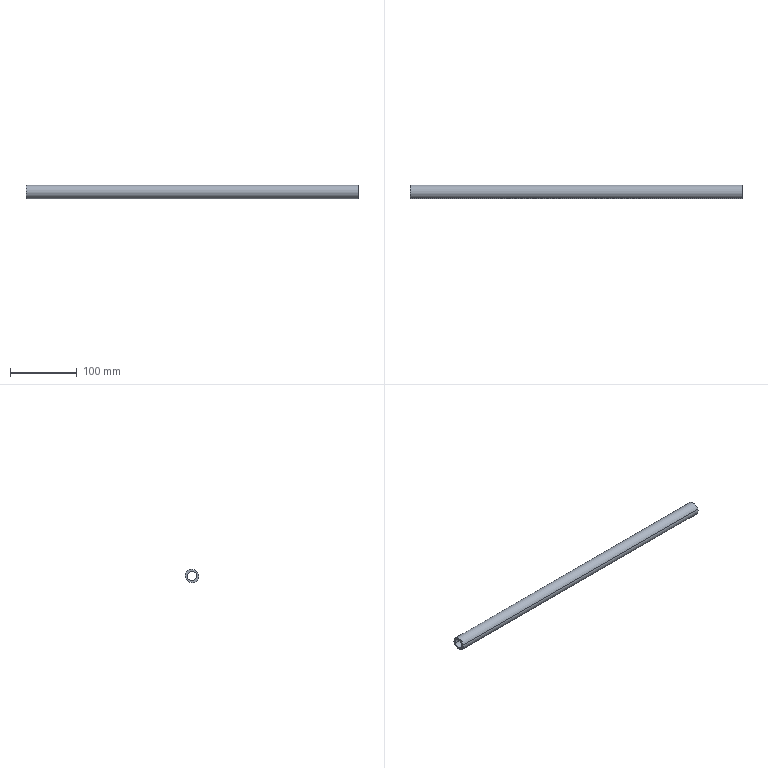Component | SolidWorks | Part9-1 | 1 solid | 6 faces | box 498 x 20 x 20 mm | volume 79790 mm3 | cylinder 4 | plane 2 | commonest cylinder face diameters 14 x2 20 x2 | material 45
build123d program:
from build123d import *

# Parameters (mm, degrees)
BOSS_EXTRUDE1_DEPTH      = 462
BOSS_EXTRUDE1_DEPTH_BACK = 36
SKETCH4_R                = 10
SKETCH5_R                = 7
CUT_EXTRUDE1_DEPTH       = 500.106


with BuildPart() as part:
    # Sketch4 → Boss-Extrude1 (new, two sides: drawn at the far end of the back side and taken through both)
    with BuildSketch(Plane.XY.offset(-BOSS_EXTRUDE1_DEPTH_BACK)):
        with Locations((16.5, -10.004)):
            Circle(SKETCH4_R)
    extrude(amount=BOSS_EXTRUDE1_DEPTH + BOSS_EXTRUDE1_DEPTH_BACK)

    # Sketch5 → Cut-Extrude1 (cut, through all)
    with BuildSketch(Plane(origin=(0, 0, -36), x_dir=(-1, 0, 0), z_dir=(0, 0, -1))):
        with Locations((-16.5, -10.004)):
            Circle(SKETCH5_R)
    extrude(amount=-CUT_EXTRUDE1_DEPTH, mode=Mode.SUBTRACT)


solid = part.part

# Placed as in the assembly
solid = solid.moved(Location((8.954, -34.996, 26.504), (0, 90, 0)))
STEP:
#1=CARTESIAN_POINT('',(18.541,-2.036,0.4706));
#2=VERTEX_POINT('',#1);
#3=CARTESIAN_POINT('',(18.541,-1.507,0.3171));
#4=VERTEX_POINT('',#3);
#5=CARTESIAN_POINT('',(18.541,-1.772,0.3939));
#6=DIRECTION('',(-1.,-0.,0.));
#7=DIRECTION('',(0.,0.9604,-0.2785));
#8=AXIS2_PLACEMENT_3D('',#5,#6,#7);
#9=CIRCLE('',#8,0.2756);
#10=EDGE_CURVE('',#2,#4,#9,.T.);
#11=ORIENTED_EDGE('',*,*,#10,.F.);
#12=CARTESIAN_POINT('',(-1.065,-2.036,0.4706));
#13=VERTEX_POINT('',#12);
#14=CARTESIAN_POINT('',(18.541,-2.036,0.4706));
#15=DIRECTION('',(-1.,-0.,0.));
#16=VECTOR('',#15,39.37);
#17=LINE('',#14,#16);
#18=EDGE_CURVE('',#2,#13,#17,.T.);
#19=ORIENTED_EDGE('',*,*,#18,.T.);
#20=CARTESIAN_POINT('',(-1.065,-1.507,0.3171));
#21=VERTEX_POINT('',#20);
#22=CARTESIAN_POINT('',(-1.065,-1.772,0.3939));
#23=DIRECTION('',(-1.,-0.,0.));
#24=DIRECTION('',(0.,0.9604,-0.2785));
#25=AXIS2_PLACEMENT_3D('',#22,#23,#24);
#26=CIRCLE('',#25,0.2756);
#27=EDGE_CURVE('',#13,#21,#26,.T.);
#28=ORIENTED_EDGE('',*,*,#27,.T.);
#29=CARTESIAN_POINT('',(18.541,-1.507,0.3171));
#30=DIRECTION('',(-1.,-0.,0.));
#31=VECTOR('',#30,39.37);
#32=LINE('',#29,#31);
#33=EDGE_CURVE('',#4,#21,#32,.T.);
#34=ORIENTED_EDGE('',*,*,#33,.F.);
#35=EDGE_LOOP('',(#11,#19,#28,#34));
#36=FACE_OUTER_BOUND('',#35,.T.);
#37=CARTESIAN_POINT('',(18.541,-1.772,0.3939));
#38=DIRECTION('',(-1.,-0.,0.));
#39=DIRECTION('',(0.,0.9604,-0.2785));
#40=AXIS2_PLACEMENT_3D('',#37,#38,#39);
#41=CYLINDRICAL_SURFACE('',#40,0.2756);
#42=ADVANCED_FACE('',(#36),#41,.F.);
#43=CARTESIAN_POINT('',(-1.065,-2.15,0.5035));
#44=VERTEX_POINT('',#43);
#45=CARTESIAN_POINT('',(-1.065,-1.394,0.2842));
#46=VERTEX_POINT('',#45);
#47=CARTESIAN_POINT('',(-1.065,-1.772,0.3939));
#48=DIRECTION('',(1.,0.,-0.));
#49=DIRECTION('',(0.,-0.9604,0.2785));
#50=AXIS2_PLACEMENT_3D('',#47,#48,#49);
#51=CIRCLE('',#50,0.3937);
#52=EDGE_CURVE('',#44,#46,#51,.T.);
#53=ORIENTED_EDGE('',*,*,#52,.T.);
#54=CARTESIAN_POINT('',(18.541,-1.394,0.2842));
#55=VERTEX_POINT('',#54);
#56=CARTESIAN_POINT('',(-1.065,-1.394,0.2842));
#57=DIRECTION('',(1.,0.,-0.));
#58=VECTOR('',#57,39.37);
#59=LINE('',#56,#58);
#60=EDGE_CURVE('',#46,#55,#59,.T.);
#61=ORIENTED_EDGE('',*,*,#60,.T.);
#62=CARTESIAN_POINT('',(18.541,-2.15,0.5035));
#63=VERTEX_POINT('',#62);
#64=CARTESIAN_POINT('',(18.541,-1.772,0.3939));
#65=DIRECTION('',(1.,0.,-0.));
#66=DIRECTION('',(0.,-0.9604,0.2785));
#67=AXIS2_PLACEMENT_3D('',#64,#65,#66);
#68=CIRCLE('',#67,0.3937);
#69=EDGE_CURVE('',#63,#55,#68,.T.);
#70=ORIENTED_EDGE('',*,*,#69,.F.);
#71=CARTESIAN_POINT('',(-1.065,-2.15,0.5035));
#72=DIRECTION('',(1.,0.,-0.));
#73=VECTOR('',#72,39.37);
#74=LINE('',#71,#73);
#75=EDGE_CURVE('',#44,#63,#74,.T.);
#76=ORIENTED_EDGE('',*,*,#75,.F.);
#77=EDGE_LOOP('',(#53,#61,#70,#76));
#78=FACE_OUTER_BOUND('',#77,.T.);
#79=CARTESIAN_POINT('',(-1.065,-1.772,0.3939));
#80=DIRECTION('',(1.,0.,-0.));
#81=DIRECTION('',(0.,-0.9604,0.2785));
#82=AXIS2_PLACEMENT_3D('',#79,#80,#81);
#83=CYLINDRICAL_SURFACE('',#82,0.3937);
#84=ADVANCED_FACE('',(#78),#83,.T.);
#85=ORIENTED_EDGE('',*,*,#60,.F.);
#86=CARTESIAN_POINT('',(-1.065,-1.772,0.3939));
#87=DIRECTION('',(1.,0.,-0.));
#88=DIRECTION('',(0.,-0.9604,0.2785));
#89=AXIS2_PLACEMENT_3D('',#86,#87,#88);
#90=CIRCLE('',#89,0.3937);
#91=EDGE_CURVE('',#46,#44,#90,.T.);
#92=ORIENTED_EDGE('',*,*,#91,.T.);
#93=ORIENTED_EDGE('',*,*,#75,.T.);
#94=CARTESIAN_POINT('',(18.541,-1.772,0.3939));
#95=DIRECTION('',(1.,0.,-0.));
#96=DIRECTION('',(0.,-0.9604,0.2785));
#97=AXIS2_PLACEMENT_3D('',#94,#95,#96);
#98=CIRCLE('',#97,0.3937);
#99=EDGE_CURVE('',#55,#63,#98,.T.);
#100=ORIENTED_EDGE('',*,*,#99,.F.);
#101=EDGE_LOOP('',(#85,#92,#93,#100));
#102=FACE_OUTER_BOUND('',#101,.T.);
#103=CARTESIAN_POINT('',(-1.065,-1.772,0.3939));
#104=DIRECTION('',(1.,0.,-0.));
#105=DIRECTION('',(0.,-0.9604,0.2785));
#106=AXIS2_PLACEMENT_3D('',#103,#104,#105);
#107=CYLINDRICAL_SURFACE('',#106,0.3937);
#108=ADVANCED_FACE('',(#102),#107,.T.);
#109=CARTESIAN_POINT('',(-1.065,-1.772,0.3939));
#110=DIRECTION('',(-1.,-0.,0.));
#111=DIRECTION('',(0.,0.9604,-0.2785));
#112=AXIS2_PLACEMENT_3D('',#109,#110,#111);
#113=CIRCLE('',#112,0.2756);
#114=EDGE_CURVE('',#21,#13,#113,.T.);
#115=ORIENTED_EDGE('',*,*,#114,.F.);
#116=ORIENTED_EDGE('',*,*,#27,.F.);
#117=EDGE_LOOP('',(#115,#116));
#118=FACE_BOUND('',#117,.T.);
#119=ORIENTED_EDGE('',*,*,#52,.F.);
#120=ORIENTED_EDGE('',*,*,#91,.F.);
#121=EDGE_LOOP('',(#119,#120));
#122=FACE_OUTER_BOUND('',#121,.T.);
#123=CARTESIAN_POINT('',(-1.065,-1.772,0.3939));
#124=DIRECTION('',(1.,0.,-0.));
#125=DIRECTION('',(0.,-0.9604,0.2785));
#126=AXIS2_PLACEMENT_3D('',#123,#124,#125);
#127=PLANE('',#126);
#128=ADVANCED_FACE('',(#118,#122),#127,.F.);
#129=CARTESIAN_POINT('',(18.541,-1.772,0.3939));
#130=DIRECTION('',(-1.,-0.,0.));
#131=DIRECTION('',(0.,0.9604,-0.2785));
#132=AXIS2_PLACEMENT_3D('',#129,#130,#131);
#133=CIRCLE('',#132,0.2756);
#134=EDGE_CURVE('',#4,#2,#133,.T.);
#135=ORIENTED_EDGE('',*,*,#134,.T.);
#136=ORIENTED_EDGE('',*,*,#10,.T.);
#137=EDGE_LOOP('',(#135,#136));
#138=FACE_BOUND('',#137,.T.);
#139=ORIENTED_EDGE('',*,*,#69,.T.);
#140=ORIENTED_EDGE('',*,*,#99,.T.);
#141=EDGE_LOOP('',(#139,#140));
#142=FACE_OUTER_BOUND('',#141,.T.);
#143=CARTESIAN_POINT('',(18.541,-1.772,0.3939));
#144=DIRECTION('',(1.,0.,-0.));
#145=DIRECTION('',(0.,-0.9604,0.2785));
#146=AXIS2_PLACEMENT_3D('',#143,#144,#145);
#147=PLANE('',#146);
#148=ADVANCED_FACE('',(#138,#142),#147,.T.);
#149=ORIENTED_EDGE('',*,*,#18,.F.);
#150=ORIENTED_EDGE('',*,*,#134,.F.);
#151=ORIENTED_EDGE('',*,*,#33,.T.);
#152=ORIENTED_EDGE('',*,*,#114,.T.);
#153=EDGE_LOOP('',(#149,#150,#151,#152));
#154=FACE_OUTER_BOUND('',#153,.T.);
#155=CARTESIAN_POINT('',(18.541,-1.772,0.3939));
#156=DIRECTION('',(-1.,-0.,0.));
#157=DIRECTION('',(0.,0.9604,-0.2785));
#158=AXIS2_PLACEMENT_3D('',#155,#156,#157);
#159=CYLINDRICAL_SURFACE('',#158,0.2756);
#160=ADVANCED_FACE('',(#154),#159,.F.);
#161=CLOSED_SHELL('',(#42,#84,#108,#128,#148,#160));
#162=MANIFOLD_SOLID_BREP('',#161);
#163=CARTESIAN_POINT('',(0.,0.,0.));
#164=DIRECTION('',(0.,0.,1.));
#165=DIRECTION('',(1.,0.,0.));
#166=AXIS2_PLACEMENT_3D('',#163,#164,#165);
#167=(LENGTH_UNIT()NAMED_UNIT(*)SI_UNIT($,.METRE.));
#168=LENGTH_MEASURE_WITH_UNIT(LENGTH_MEASURE(0.0254),#167);
#169=DIMENSIONAL_EXPONENTS(1.,0.,0.,0.,0.,0.,0.);
#170=(CONVERSION_BASED_UNIT('',#168)LENGTH_UNIT()NAMED_UNIT(#169));
#171=UNCERTAINTY_MEASURE_WITH_UNIT(LENGTH_MEASURE(0.00001),#170,'','');
#172=(NAMED_UNIT(*)PLANE_ANGLE_UNIT()SI_UNIT($,.RADIAN.));
#173=(NAMED_UNIT(*)SI_UNIT($,.STERADIAN.)SOLID_ANGLE_UNIT());
#174=(GEOMETRIC_REPRESENTATION_CONTEXT(3)GLOBAL_UNCERTAINTY_ASSIGNED_CONTEXT((#171))GLOBAL_UNIT_ASSIGNED_CONTEXT((#170,#172,#173))REPRESENTATION_CONTEXT('',''));
#175=ADVANCED_BREP_SHAPE_REPRESENTATION('',(#162,#166),#174);
#176=COLOUR_RGB('',0.7922,0.8196,0.9333);
#177=FILL_AREA_STYLE_COLOUR('',#176);
#178=FILL_AREA_STYLE('',(#177));
#179=SURFACE_STYLE_FILL_AREA(#178);
#180=SURFACE_SIDE_STYLE('',(#179));
#181=SURFACE_STYLE_USAGE(.BOTH.,#180);
#182=PRESENTATION_STYLE_ASSIGNMENT((#181));
#183=STYLED_ITEM('',(#182),#162);
#184=(LENGTH_UNIT()NAMED_UNIT(*)SI_UNIT($,.METRE.));
#185=LENGTH_MEASURE_WITH_UNIT(LENGTH_MEASURE(0.0254),#184);
#186=DIMENSIONAL_EXPONENTS(1.,0.,0.,0.,0.,0.,0.);
#187=(CONVERSION_BASED_UNIT('',#185)LENGTH_UNIT()NAMED_UNIT(#186));
#188=UNCERTAINTY_MEASURE_WITH_UNIT(LENGTH_MEASURE(0.00001),#187,'','');
#189=(NAMED_UNIT(*)PLANE_ANGLE_UNIT()SI_UNIT($,.RADIAN.));
#190=(NAMED_UNIT(*)SI_UNIT($,.STERADIAN.)SOLID_ANGLE_UNIT());
#191=(GEOMETRIC_REPRESENTATION_CONTEXT(3)GLOBAL_UNCERTAINTY_ASSIGNED_CONTEXT((#188))GLOBAL_UNIT_ASSIGNED_CONTEXT((#187,#189,#190))REPRESENTATION_CONTEXT('',''));
#192=MECHANICAL_DESIGN_GEOMETRIC_PRESENTATION_REPRESENTATION('',(#183),#191);
#193=PRESENTATION_LAYER_ASSIGNMENT('','',(#183));